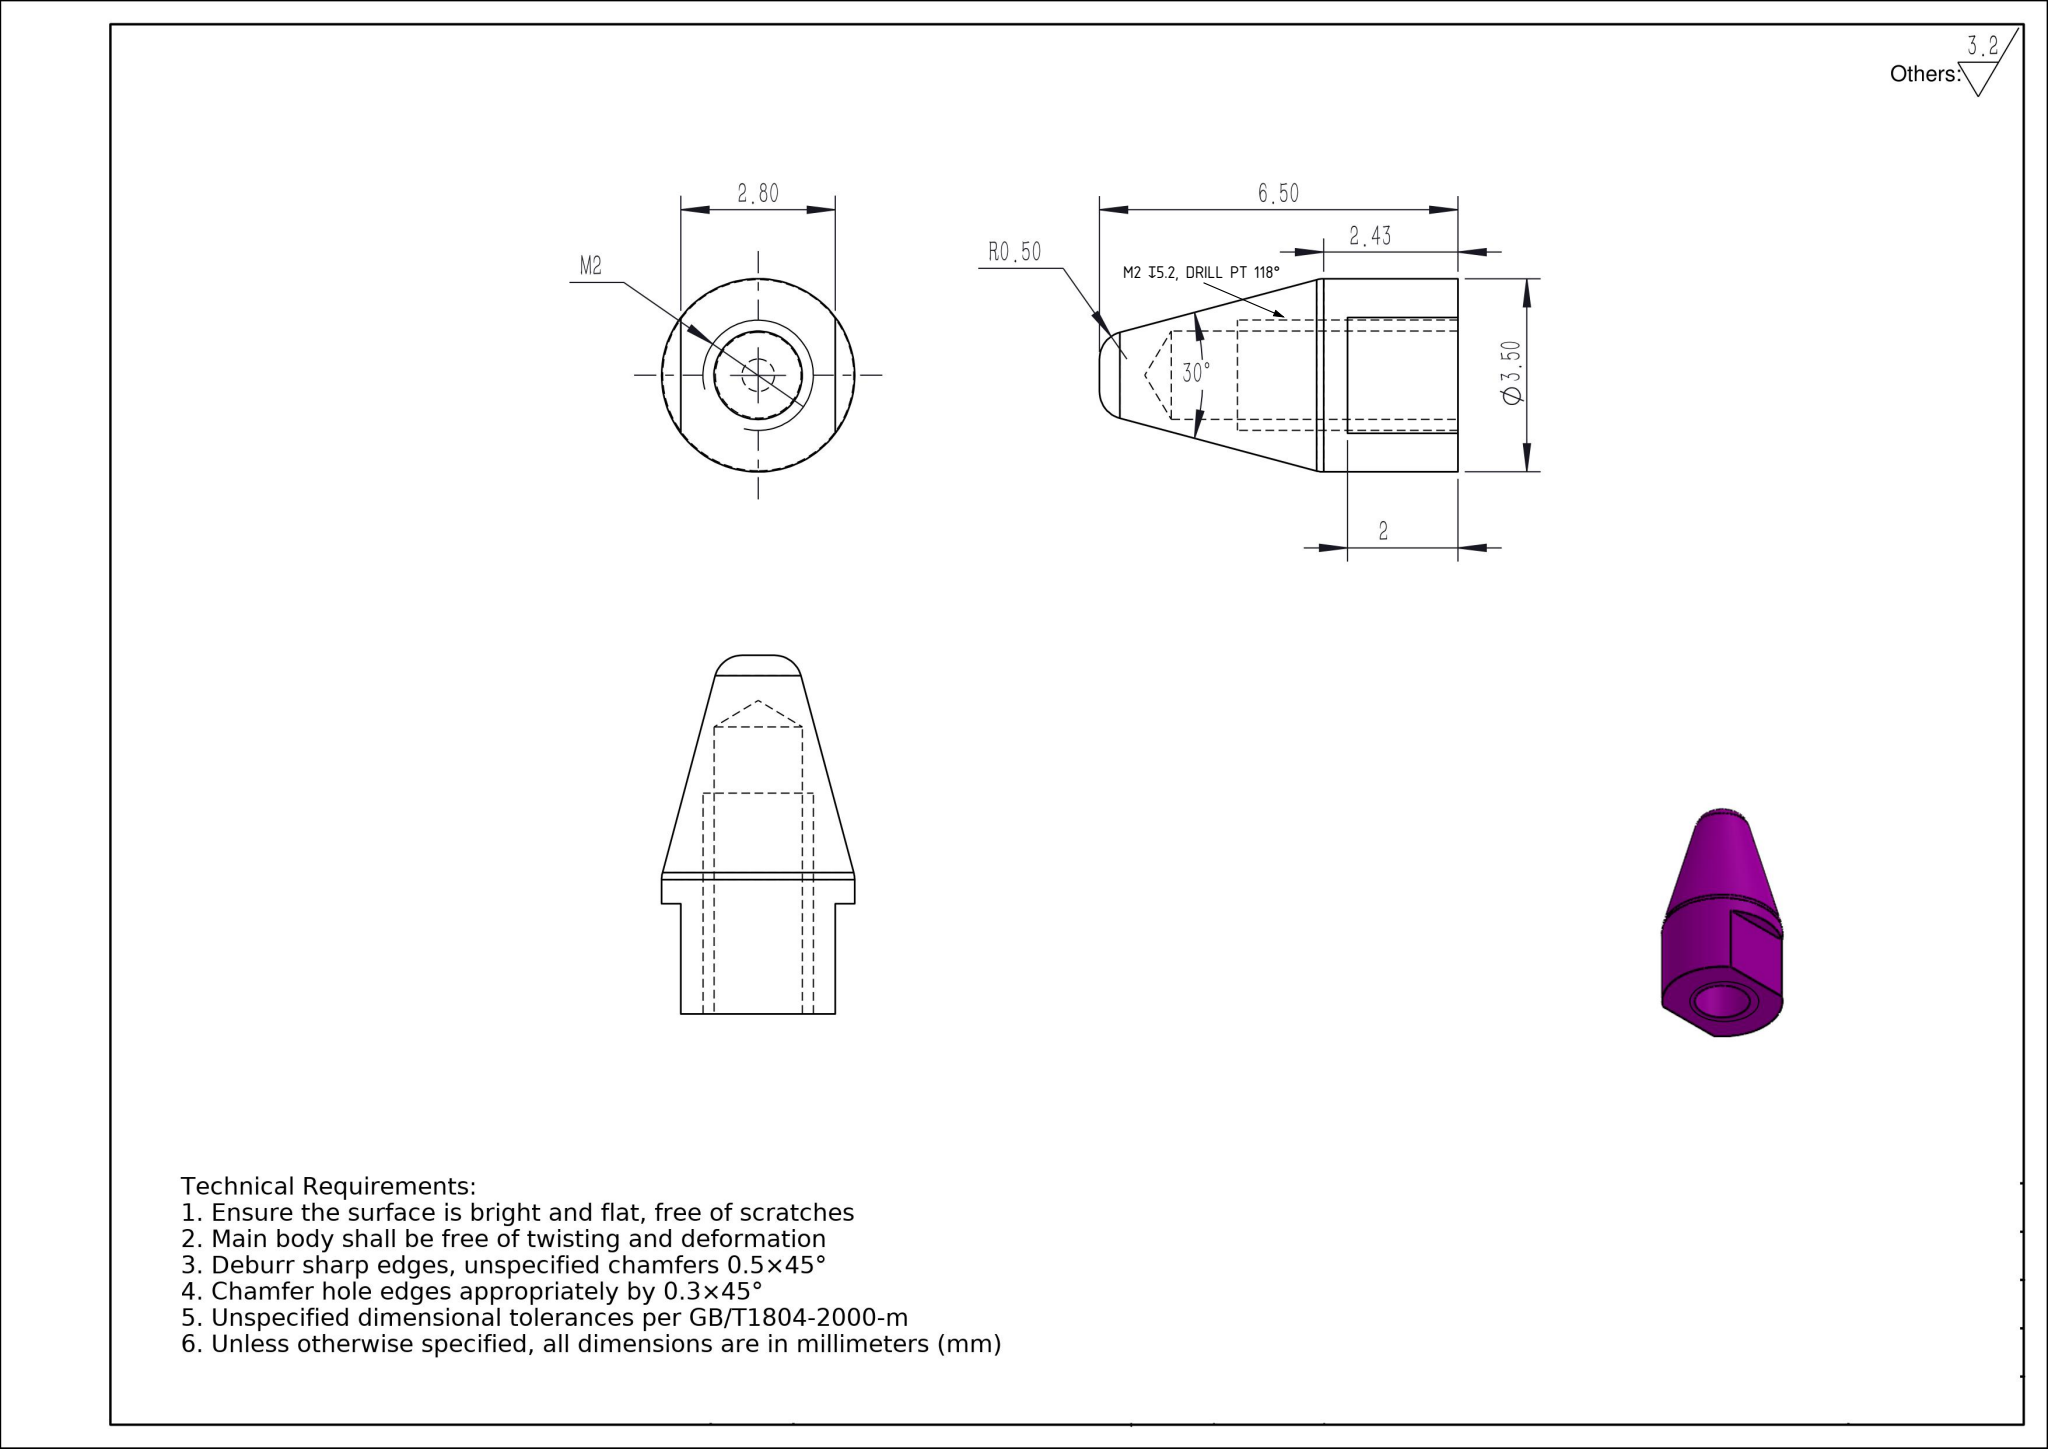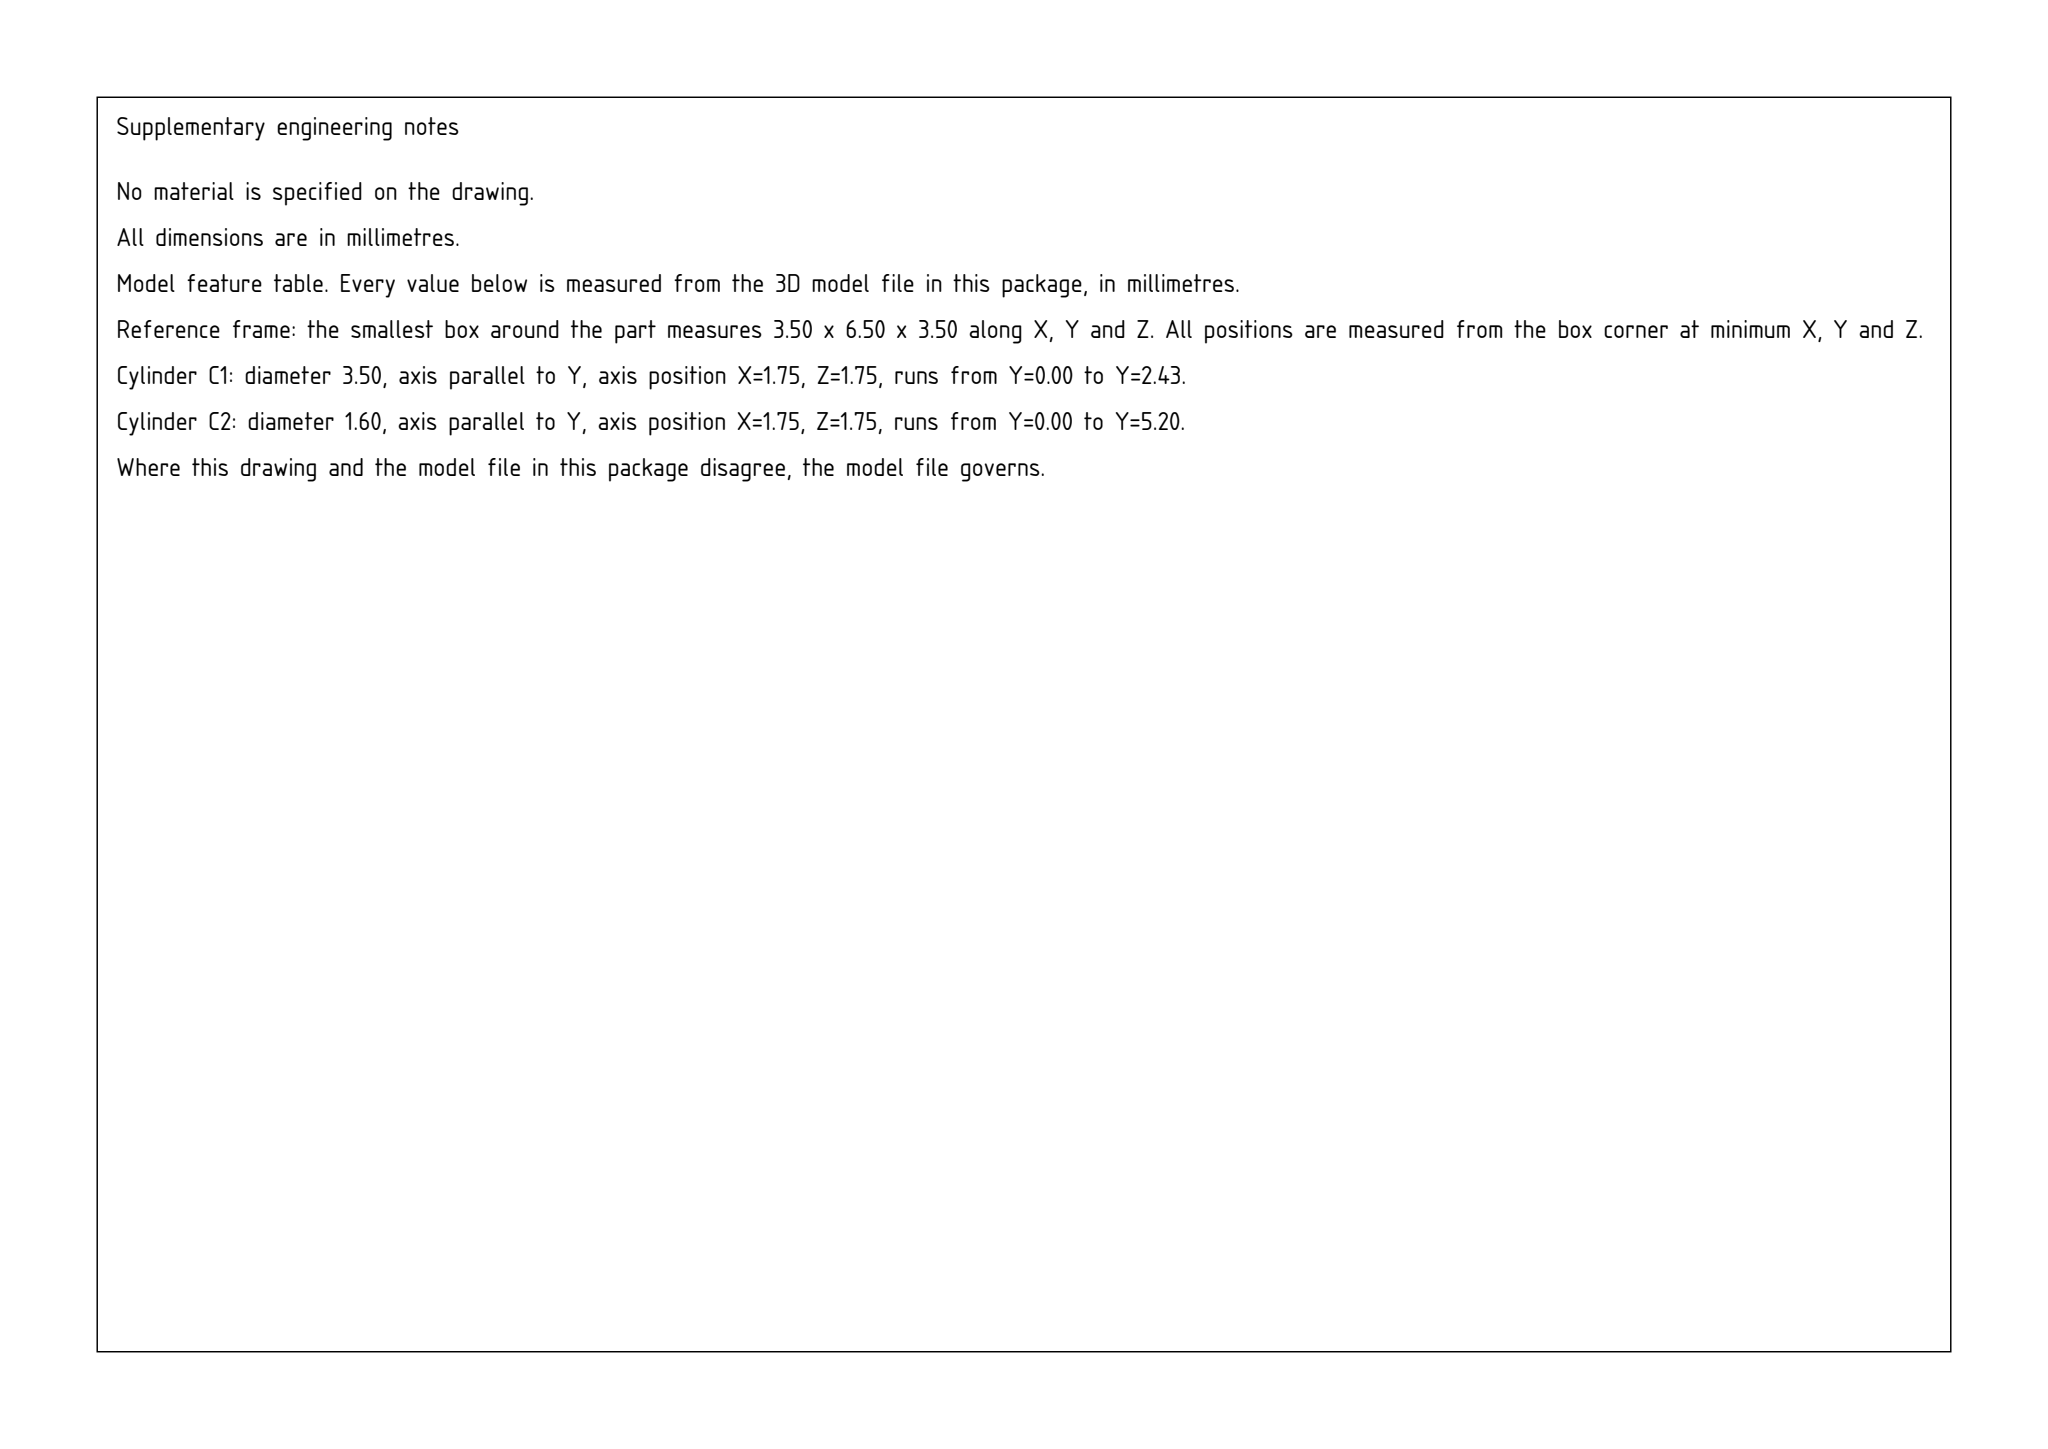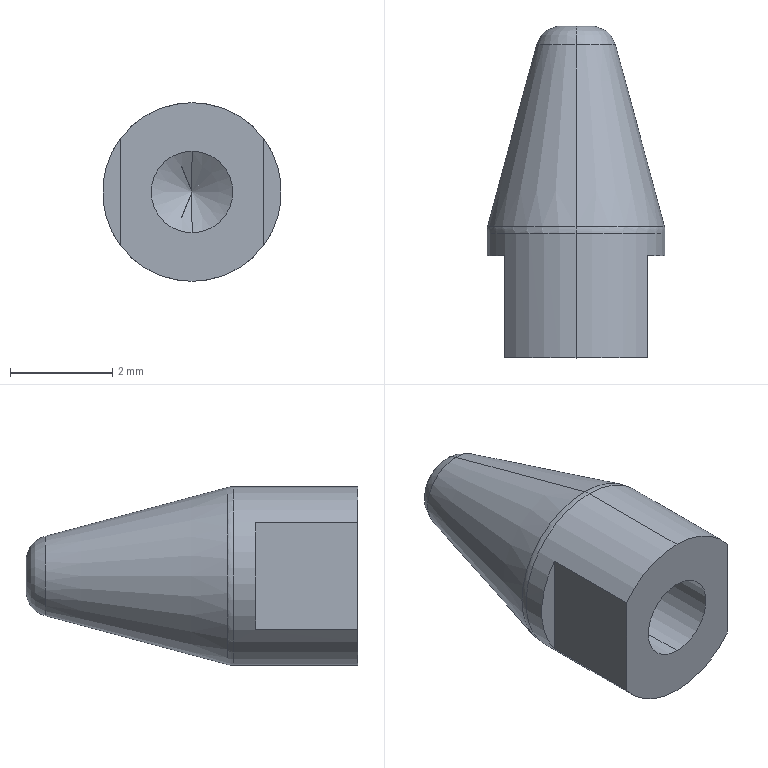Part | SolidWorks | mm | 1 solid | 18 faces | box 3.5 x 6.5 x 3.5 mm | volume 31 mm3 | plane 6 | cylinder 4 | cone 4 | torus 4 | commonest cylinder face diameters 1.6 x2 3.5 x2
Drawing notes:
M2 DP 5.2 FROM Ø3.5 END FACE; DRILL PT 118° | from the solid: cylinder dia 1.6, axis y, length 5.2 from y=6.5 face; cone incl angle 118° ref dia 1.6
build123d program:
from build123d import *

# Parameters (mm, degrees)
SKETCH1_R             = 1.75
BOSS_EXTRUDE1_DEPTH   = 6.5
CHAMFER1_SIZE         = 4
CHAMFER1_SIZE2        = 1.072
FILLET2_R             = 0.5
M2_TAPPED_HOLE1_D     = 1.6
M2_TAPPED_HOLE1_DEPTH = 5.2
M2_TAPPED_HOLE1_TIP   = 0.4807
SKETCH4_OUTSIDE_W     = 7.134
SKETCH4_OUTSIDE_H     = 7.134
SKETCH4_OUTSIDE_W_2   = 2.8
SKETCH4_OUTSIDE_H_2   = 5.076
CUT_EXTRUDE1_DEPTH    = 2


with BuildPart() as part:
    # Sketch1 → Boss-Extrude1 (new body)
    with BuildSketch(Plane(origin=(0, 0, 0), x_dir=(1, 0, 0), z_dir=(0, 1, 0))):
        with Locations(Location((0, 0, 0), (0, 0, 90))):
            Circle(SKETCH1_R)
    extrude(amount=BOSS_EXTRUDE1_DEPTH)

    # Chamfer1
    chamfer1_edges = [part.edges().sort_by_distance(p)[0] for p in [
        (0, 6.5, 1.75),
    ]]
    chamfer1_side = [part.faces().sort_by_distance(p)[0] for p in [
        (0, 3.25, 1.75),
    ]]
    chamfer(chamfer1_edges, length=CHAMFER1_SIZE, length2=CHAMFER1_SIZE2, reference=chamfer1_side[0])

    # Fillet2
    fillet2_edges = [part.edges().sort_by_distance(p)[0] for p in [
        (0, 6.5, 0.6782),
        (0, 2.5, 1.75),
    ]]
    fillet(fillet2_edges, radius=FILLET2_R)

    # M2 Tapped Hole1
    with Locations(Plane(origin=(0, 0, 0), x_dir=(-1, 0, 0), z_dir=(0, -1, 0))):
        with Locations((0, 0)):
            Hole(M2_TAPPED_HOLE1_D / 2, depth=M2_TAPPED_HOLE1_DEPTH)
            with Locations((0, 0, -(M2_TAPPED_HOLE1_DEPTH + M2_TAPPED_HOLE1_TIP / 2))):  # 118° drill point
                Cone(0, M2_TAPPED_HOLE1_D / 2, M2_TAPPED_HOLE1_TIP, mode=Mode.SUBTRACT)

    # Sketch4 outside → Cut-Extrude1 (cut)
    with BuildSketch(Plane.XZ):
        Rectangle(SKETCH4_OUTSIDE_W, SKETCH4_OUTSIDE_H)
        Rectangle(SKETCH4_OUTSIDE_W_2, SKETCH4_OUTSIDE_H_2, mode=Mode.SUBTRACT)
    extrude(amount=-CUT_EXTRUDE1_DEPTH, mode=Mode.SUBTRACT)


solid = part.part